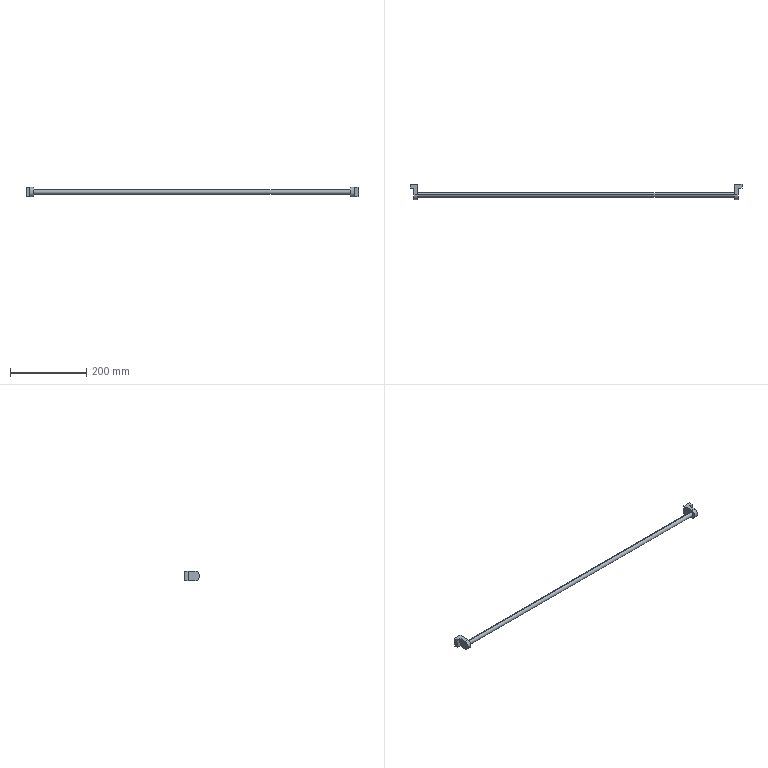Component | SolidWorks | D014-1 | 2 solids | 22 faces | box 869 x 40 x 25 mm | volume 117416 mm3 | plane 16 | cylinder 6 | commonest cylinder face diameters 12 x4 25 x2
build123d program:
from build123d import *

# Parameters (mm, degrees)
SKETCH1_W           = 40
SKETCH1_H           = 25
BOSS_EXTRUDE1_DEPTH = 10
FILLET1_RADIUS      = 12.5
FILLET1_LENGTH      = 10
SKETCH2_R           = 6
CUT_EXTRUDE1_DEPTH  = 2
SKETCH3_R           = 6
BOSS_EXTRUDE2_DEPTH = 831
BOSS_EXTRUDE3_START = 10
BOSS_EXTRUDE3_DEPTH = 10
SKETCH5_W           = 25
SKETCH5_H           = 10
BOSS_EXTRUDE4_DEPTH = 10
SKETCH6_W           = 25
SKETCH6_H           = 10
BOSS_EXTRUDE5_DEPTH = 10


with BuildPart() as part:
    # Sketch1 → Boss-Extrude1 (new body)
    with BuildSketch(Plane(origin=(0, 0, 0), x_dir=(1, 0, 0), z_dir=(0, 1, 0))):
        with Locations((20, 12.5)):
            Rectangle(SKETCH1_W, SKETCH1_H)
    extrude(amount=BOSS_EXTRUDE1_DEPTH)

    # Fillet1: full round fillet: the end face becomes a half cylinder, R = half its width
    fillet1_face = Plane((40, 5, -12.5), x_dir=(0, 1, 0), z_dir=(1, 0, 0))  # on the end face: x along it, z out of the body
    fillet1_slab = fillet1_face.offset(-FILLET1_RADIUS / 2) * Box(FILLET1_LENGTH, 2 * FILLET1_RADIUS, FILLET1_RADIUS, mode=Mode.PRIVATE)  # the body's end, R deep
    fillet1_round = Plane((27.5, 5, -12.5), x_dir=(1, 0, 0), z_dir=(0, 1, 0)) * Cylinder(FILLET1_RADIUS, FILLET1_LENGTH, mode=Mode.PRIVATE)  # its axis R under the face
    add(fillet1_slab - fillet1_round, mode=Mode.SUBTRACT)

    # Sketch2 → Cut-Extrude1 (cut)
    with BuildSketch(Plane(origin=(0, 10, 0), x_dir=(1, 0, 0), z_dir=(0, 1, 0))):
        with Locations(Location((27.5, 12.5, 0), (0, 0, 270))):
            Circle(SKETCH2_R)
    extrude(amount=-CUT_EXTRUDE1_DEPTH, mode=Mode.SUBTRACT)

    # Sketch6 → Boss-Extrude5 (add)
    with BuildSketch(Plane.ZY):
        with Locations((-12.5, -5)):
            Rectangle(SKETCH6_W, SKETCH6_H)
    extrude(amount=-BOSS_EXTRUDE5_DEPTH)


with BuildPart() as body_2:
    # Sketch3 → Boss-Extrude2 (new body)
    with BuildSketch(Plane(origin=(0, 8, 0), x_dir=(1, 0, 0), z_dir=(0, 1, 0))):
        with Locations(Location((27.5, 12.5, 0), (0, 0, 270))):
            Circle(SKETCH3_R)
    extrude(amount=BOSS_EXTRUDE2_DEPTH)

    # Sketch4 → Boss-Extrude3 (add)
    with BuildSketch(Plane(origin=(0, 839, 0), x_dir=(1, 0, 0), z_dir=(0, 1, 0)).offset(BOSS_EXTRUDE3_START)):
        with BuildLine():
            Line((0, 0), (27.5, 0))
            ThreePointArc((27.5, 0), (40, 12.5), (27.5, 25))
            Line((27.5, 25), (0, 25))
            Line((0, 25), (0, 0))
        make_face()
    extrude(amount=-BOSS_EXTRUDE3_DEPTH)

    # Sketch5 → Boss-Extrude4 (add)
    with BuildSketch(Plane.ZY):
        with Locations((-12.5, 854)):
            Rectangle(SKETCH5_W, SKETCH5_H)
    extrude(amount=-BOSS_EXTRUDE4_DEPTH)


solid = Compound([part.part, body_2.part])

# Placed as in the assembly
solid = solid.moved(Location((859, -60, -101.268), (180, 0, 90)))
STEP:
#1=COLOUR_RGB('',0.7922,0.8196,0.9333);
#2=FILL_AREA_STYLE_COLOUR('',#1);
#3=FILL_AREA_STYLE('',(#2));
#4=SURFACE_STYLE_FILL_AREA(#3);
#5=SURFACE_SIDE_STYLE('',(#4));
#6=SURFACE_STYLE_USAGE(.BOTH.,#5);
#7=PRESENTATION_STYLE_ASSIGNMENT((#6));
#8=CARTESIAN_POINT('',(33.504,-3.445,-3.259));
#9=VERTEX_POINT('',#8);
#10=CARTESIAN_POINT('',(33.504,-3.445,-3.731));
#11=VERTEX_POINT('',#10);
#12=CARTESIAN_POINT('',(33.504,-3.445,-3.495));
#13=DIRECTION('',(-1.,0.,0.));
#14=DIRECTION('',(0.,0.,-1.));
#15=AXIS2_PLACEMENT_3D('',#12,#13,#14);
#16=CIRCLE('',#15,0.2362);
#17=EDGE_CURVE('',#9,#11,#16,.T.);
#18=ORIENTED_EDGE('',*,*,#17,.F.);
#19=CARTESIAN_POINT('',(33.425,-3.445,-3.259));
#20=VERTEX_POINT('',#19);
#21=CARTESIAN_POINT('',(33.504,-3.445,-3.259));
#22=DIRECTION('',(-1.,0.,0.));
#23=VECTOR('',#22,39.37);
#24=LINE('',#21,#23);
#25=EDGE_CURVE('',#9,#20,#24,.T.);
#26=ORIENTED_EDGE('',*,*,#25,.T.);
#27=CARTESIAN_POINT('',(33.425,-3.445,-3.731));
#28=VERTEX_POINT('',#27);
#29=CARTESIAN_POINT('',(33.425,-3.445,-3.495));
#30=DIRECTION('',(-1.,0.,0.));
#31=DIRECTION('',(0.,0.,-1.));
#32=AXIS2_PLACEMENT_3D('',#29,#30,#31);
#33=CIRCLE('',#32,0.2362);
#34=EDGE_CURVE('',#20,#28,#33,.T.);
#35=ORIENTED_EDGE('',*,*,#34,.T.);
#36=CARTESIAN_POINT('',(33.504,-3.445,-3.731));
#37=DIRECTION('',(-1.,0.,0.));
#38=VECTOR('',#37,39.37);
#39=LINE('',#36,#38);
#40=EDGE_CURVE('',#11,#28,#39,.T.);
#41=ORIENTED_EDGE('',*,*,#40,.F.);
#42=EDGE_LOOP('',(#18,#26,#35,#41));
#43=FACE_OUTER_BOUND('',#42,.T.);
#44=CARTESIAN_POINT('',(33.504,-3.445,-3.495));
#45=DIRECTION('',(-1.,0.,0.));
#46=DIRECTION('',(0.,0.,-1.));
#47=AXIS2_PLACEMENT_3D('',#44,#45,#46);
#48=CYLINDRICAL_SURFACE('',#47,0.2362);
#49=ADVANCED_FACE('',(#43),#48,.F.);
#50=CARTESIAN_POINT('',(33.819,-2.756,-3.987));
#51=VERTEX_POINT('',#50);
#52=CARTESIAN_POINT('',(33.819,-3.445,-3.987));
#53=VERTEX_POINT('',#52);
#54=CARTESIAN_POINT('',(33.819,-2.362,-3.987));
#55=DIRECTION('',(-0.,-1.,-0.));
#56=VECTOR('',#55,39.37);
#57=LINE('',#54,#56);
#58=EDGE_CURVE('',#51,#53,#57,.T.);
#59=ORIENTED_EDGE('',*,*,#58,.F.);
#60=CARTESIAN_POINT('',(33.819,-2.756,-3.003));
#61=VERTEX_POINT('',#60);
#62=CARTESIAN_POINT('',(33.819,-2.756,-3.003));
#63=DIRECTION('',(0.,-0.,1.));
#64=VECTOR('',#63,39.37);
#65=LINE('',#62,#64);
#66=EDGE_CURVE('',#51,#61,#65,.T.);
#67=ORIENTED_EDGE('',*,*,#66,.T.);
#68=CARTESIAN_POINT('',(33.819,-3.445,-3.003));
#69=VERTEX_POINT('',#68);
#70=CARTESIAN_POINT('',(33.819,-2.362,-3.003));
#71=DIRECTION('',(0.,1.,0.));
#72=VECTOR('',#71,39.37);
#73=LINE('',#70,#72);
#74=EDGE_CURVE('',#69,#61,#73,.T.);
#75=ORIENTED_EDGE('',*,*,#74,.F.);
#76=CARTESIAN_POINT('',(33.819,-3.445,-3.495));
#77=DIRECTION('',(1.,-0.,-0.));
#78=DIRECTION('',(0.,-0.,1.));
#79=AXIS2_PLACEMENT_3D('',#76,#77,#78);
#80=CIRCLE('',#79,0.4921);
#81=EDGE_CURVE('',#69,#53,#80,.T.);
#82=ORIENTED_EDGE('',*,*,#81,.T.);
#83=EDGE_LOOP('',(#59,#67,#75,#82));
#84=FACE_OUTER_BOUND('',#83,.T.);
#85=CARTESIAN_POINT('',(33.819,-2.362,-3.987));
#86=DIRECTION('',(1.,-0.,-0.));
#87=DIRECTION('',(0.,-0.,1.));
#88=AXIS2_PLACEMENT_3D('',#85,#86,#87);
#89=PLANE('',#88);
#90=ADVANCED_FACE('',(#84),#89,.T.);
#91=CARTESIAN_POINT('',(33.425,-3.445,-3.987));
#92=VERTEX_POINT('',#91);
#93=CARTESIAN_POINT('',(33.425,-3.445,-3.987));
#94=DIRECTION('',(-1.,0.,0.));
#95=VECTOR('',#94,39.37);
#96=LINE('',#93,#95);
#97=EDGE_CURVE('',#53,#92,#96,.T.);
#98=ORIENTED_EDGE('',*,*,#97,.F.);
#99=ORIENTED_EDGE('',*,*,#81,.F.);
#100=CARTESIAN_POINT('',(33.425,-3.445,-3.003));
#101=VERTEX_POINT('',#100);
#102=CARTESIAN_POINT('',(33.425,-3.445,-3.003));
#103=DIRECTION('',(1.,-0.,-0.));
#104=VECTOR('',#103,39.37);
#105=LINE('',#102,#104);
#106=EDGE_CURVE('',#101,#69,#105,.T.);
#107=ORIENTED_EDGE('',*,*,#106,.F.);
#108=CARTESIAN_POINT('',(33.425,-3.445,-3.495));
#109=DIRECTION('',(-1.,0.,0.));
#110=DIRECTION('',(0.,-0.,1.));
#111=AXIS2_PLACEMENT_3D('',#108,#109,#110);
#112=CIRCLE('',#111,0.4921);
#113=EDGE_CURVE('',#92,#101,#112,.T.);
#114=ORIENTED_EDGE('',*,*,#113,.F.);
#115=EDGE_LOOP('',(#98,#99,#107,#114));
#116=FACE_OUTER_BOUND('',#115,.T.);
#117=CARTESIAN_POINT('',(33.819,-3.445,-3.495));
#118=DIRECTION('',(1.,-0.,-0.));
#119=DIRECTION('',(0.,-0.,1.));
#120=AXIS2_PLACEMENT_3D('',#117,#118,#119);
#121=CYLINDRICAL_SURFACE('',#120,0.4921);
#122=ADVANCED_FACE('',(#116),#121,.T.);
#123=CARTESIAN_POINT('',(33.425,-2.362,-3.003));
#124=VERTEX_POINT('',#123);
#125=CARTESIAN_POINT('',(34.213,-2.362,-3.003));
#126=VERTEX_POINT('',#125);
#127=CARTESIAN_POINT('',(33.425,-2.362,-3.003));
#128=DIRECTION('',(1.,-0.,-0.));
#129=VECTOR('',#128,39.37);
#130=LINE('',#127,#129);
#131=EDGE_CURVE('',#124,#126,#130,.T.);
#132=ORIENTED_EDGE('',*,*,#131,.T.);
#133=CARTESIAN_POINT('',(34.213,-2.362,-3.987));
#134=VERTEX_POINT('',#133);
#135=CARTESIAN_POINT('',(34.213,-2.362,-3.003));
#136=DIRECTION('',(-0.,0.,-1.));
#137=VECTOR('',#136,39.37);
#138=LINE('',#135,#137);
#139=EDGE_CURVE('',#126,#134,#138,.T.);
#140=ORIENTED_EDGE('',*,*,#139,.T.);
#141=CARTESIAN_POINT('',(33.425,-2.362,-3.987));
#142=VERTEX_POINT('',#141);
#143=CARTESIAN_POINT('',(33.425,-2.362,-3.987));
#144=DIRECTION('',(1.,-0.,-0.));
#145=VECTOR('',#144,39.37);
#146=LINE('',#143,#145);
#147=EDGE_CURVE('',#142,#134,#146,.T.);
#148=ORIENTED_EDGE('',*,*,#147,.F.);
#149=CARTESIAN_POINT('',(33.425,-2.362,-3.987));
#150=DIRECTION('',(-0.,0.,-1.));
#151=VECTOR('',#150,39.37);
#152=LINE('',#149,#151);
#153=EDGE_CURVE('',#124,#142,#152,.T.);
#154=ORIENTED_EDGE('',*,*,#153,.F.);
#155=EDGE_LOOP('',(#132,#140,#148,#154));
#156=FACE_OUTER_BOUND('',#155,.T.);
#157=CARTESIAN_POINT('',(33.425,-2.362,-3.987));
#158=DIRECTION('',(-0.,-1.,-0.));
#159=DIRECTION('',(0.,-0.,1.));
#160=AXIS2_PLACEMENT_3D('',#157,#158,#159);
#161=PLANE('',#160);
#162=ADVANCED_FACE('',(#156),#161,.F.);
#163=ORIENTED_EDGE('',*,*,#147,.T.);
#164=CARTESIAN_POINT('',(34.213,-2.756,-3.987));
#165=VERTEX_POINT('',#164);
#166=CARTESIAN_POINT('',(34.213,-2.756,-3.987));
#167=DIRECTION('',(0.,1.,0.));
#168=VECTOR('',#167,39.37);
#169=LINE('',#166,#168);
#170=EDGE_CURVE('',#165,#134,#169,.T.);
#171=ORIENTED_EDGE('',*,*,#170,.F.);
#172=CARTESIAN_POINT('',(33.819,-2.756,-3.987));
#173=DIRECTION('',(-1.,0.,0.));
#174=VECTOR('',#173,39.37);
#175=LINE('',#172,#174);
#176=EDGE_CURVE('',#165,#51,#175,.T.);
#177=ORIENTED_EDGE('',*,*,#176,.T.);
#178=ORIENTED_EDGE('',*,*,#58,.T.);
#179=ORIENTED_EDGE('',*,*,#97,.T.);
#180=CARTESIAN_POINT('',(33.425,-2.362,-3.987));
#181=DIRECTION('',(-0.,-1.,-0.));
#182=VECTOR('',#181,39.37);
#183=LINE('',#180,#182);
#184=EDGE_CURVE('',#142,#92,#183,.T.);
#185=ORIENTED_EDGE('',*,*,#184,.F.);
#186=EDGE_LOOP('',(#163,#171,#177,#178,#179,#185));
#187=FACE_OUTER_BOUND('',#186,.T.);
#188=CARTESIAN_POINT('',(33.425,-2.362,-3.987));
#189=DIRECTION('',(0.,-0.,1.));
#190=DIRECTION('',(0.,1.,0.));
#191=AXIS2_PLACEMENT_3D('',#188,#189,#190);
#192=PLANE('',#191);
#193=ADVANCED_FACE('',(#187),#192,.F.);
#194=CARTESIAN_POINT('',(33.425,-2.362,-3.003));
#195=DIRECTION('',(0.,1.,0.));
#196=VECTOR('',#195,39.37);
#197=LINE('',#194,#196);
#198=EDGE_CURVE('',#101,#124,#197,.T.);
#199=ORIENTED_EDGE('',*,*,#198,.F.);
#200=ORIENTED_EDGE('',*,*,#106,.T.);
#201=ORIENTED_EDGE('',*,*,#74,.T.);
#202=CARTESIAN_POINT('',(34.213,-2.756,-3.003));
#203=VERTEX_POINT('',#202);
#204=CARTESIAN_POINT('',(33.819,-2.756,-3.003));
#205=DIRECTION('',(1.,-0.,-0.));
#206=VECTOR('',#205,39.37);
#207=LINE('',#204,#206);
#208=EDGE_CURVE('',#61,#203,#207,.T.);
#209=ORIENTED_EDGE('',*,*,#208,.T.);
#210=CARTESIAN_POINT('',(34.213,-2.756,-3.003));
#211=DIRECTION('',(0.,1.,0.));
#212=VECTOR('',#211,39.37);
#213=LINE('',#210,#212);
#214=EDGE_CURVE('',#203,#126,#213,.T.);
#215=ORIENTED_EDGE('',*,*,#214,.T.);
#216=ORIENTED_EDGE('',*,*,#131,.F.);
#217=EDGE_LOOP('',(#199,#200,#201,#209,#215,#216));
#218=FACE_OUTER_BOUND('',#217,.T.);
#219=CARTESIAN_POINT('',(33.425,-2.362,-3.003));
#220=DIRECTION('',(-0.,0.,-1.));
#221=DIRECTION('',(-0.,-1.,-0.));
#222=AXIS2_PLACEMENT_3D('',#219,#220,#221);
#223=PLANE('',#222);
#224=ADVANCED_FACE('',(#218),#223,.F.);
#225=CARTESIAN_POINT('',(33.425,-3.445,-3.495));
#226=DIRECTION('',(-1.,0.,0.));
#227=DIRECTION('',(0.,0.,-1.));
#228=AXIS2_PLACEMENT_3D('',#225,#226,#227);
#229=CIRCLE('',#228,0.2362);
#230=EDGE_CURVE('',#28,#20,#229,.T.);
#231=ORIENTED_EDGE('',*,*,#230,.F.);
#232=ORIENTED_EDGE('',*,*,#34,.F.);
#233=EDGE_LOOP('',(#231,#232));
#234=FACE_BOUND('',#233,.T.);
#235=ORIENTED_EDGE('',*,*,#184,.T.);
#236=ORIENTED_EDGE('',*,*,#113,.T.);
#237=ORIENTED_EDGE('',*,*,#198,.T.);
#238=ORIENTED_EDGE('',*,*,#153,.T.);
#239=EDGE_LOOP('',(#235,#236,#237,#238));
#240=FACE_OUTER_BOUND('',#239,.T.);
#241=CARTESIAN_POINT('',(33.425,-2.362,-3.987));
#242=DIRECTION('',(1.,-0.,-0.));
#243=DIRECTION('',(0.,-0.,1.));
#244=AXIS2_PLACEMENT_3D('',#241,#242,#243);
#245=PLANE('',#244);
#246=ADVANCED_FACE('',(#234,#240),#245,.F.);
#247=ORIENTED_EDGE('',*,*,#25,.F.);
#248=CARTESIAN_POINT('',(33.504,-3.445,-3.495));
#249=DIRECTION('',(-1.,0.,0.));
#250=DIRECTION('',(0.,0.,-1.));
#251=AXIS2_PLACEMENT_3D('',#248,#249,#250);
#252=CIRCLE('',#251,0.2362);
#253=EDGE_CURVE('',#11,#9,#252,.T.);
#254=ORIENTED_EDGE('',*,*,#253,.F.);
#255=ORIENTED_EDGE('',*,*,#40,.T.);
#256=ORIENTED_EDGE('',*,*,#230,.T.);
#257=EDGE_LOOP('',(#247,#254,#255,#256));
#258=FACE_OUTER_BOUND('',#257,.T.);
#259=CARTESIAN_POINT('',(33.504,-3.445,-3.495));
#260=DIRECTION('',(-1.,0.,0.));
#261=DIRECTION('',(0.,0.,-1.));
#262=AXIS2_PLACEMENT_3D('',#259,#260,#261);
#263=CYLINDRICAL_SURFACE('',#262,0.2362);
#264=ADVANCED_FACE('',(#258),#263,.F.);
#265=ORIENTED_EDGE('',*,*,#253,.T.);
#266=ORIENTED_EDGE('',*,*,#17,.T.);
#267=EDGE_LOOP('',(#265,#266));
#268=FACE_OUTER_BOUND('',#267,.T.);
#269=CARTESIAN_POINT('',(33.504,-3.445,-3.495));
#270=DIRECTION('',(-1.,0.,0.));
#271=DIRECTION('',(-0.,0.,-1.));
#272=AXIS2_PLACEMENT_3D('',#269,#270,#271);
#273=PLANE('',#272);
#274=ADVANCED_FACE('',(#268),#273,.T.);
#275=ORIENTED_EDGE('',*,*,#139,.F.);
#276=ORIENTED_EDGE('',*,*,#214,.F.);
#277=CARTESIAN_POINT('',(34.213,-2.756,-3.003));
#278=DIRECTION('',(-0.,0.,-1.));
#279=VECTOR('',#278,39.37);
#280=LINE('',#277,#279);
#281=EDGE_CURVE('',#203,#165,#280,.T.);
#282=ORIENTED_EDGE('',*,*,#281,.T.);
#283=ORIENTED_EDGE('',*,*,#170,.T.);
#284=EDGE_LOOP('',(#275,#276,#282,#283));
#285=FACE_OUTER_BOUND('',#284,.T.);
#286=CARTESIAN_POINT('',(34.213,-2.756,-3.003));
#287=DIRECTION('',(1.,-0.,-0.));
#288=DIRECTION('',(0.,-0.,1.));
#289=AXIS2_PLACEMENT_3D('',#286,#287,#288);
#290=PLANE('',#289);
#291=ADVANCED_FACE('',(#285),#290,.T.);
#292=ORIENTED_EDGE('',*,*,#208,.F.);
#293=ORIENTED_EDGE('',*,*,#66,.F.);
#294=ORIENTED_EDGE('',*,*,#176,.F.);
#295=ORIENTED_EDGE('',*,*,#281,.F.);
#296=EDGE_LOOP('',(#292,#293,#294,#295));
#297=FACE_OUTER_BOUND('',#296,.T.);
#298=CARTESIAN_POINT('',(33.819,-2.756,-3.987));
#299=DIRECTION('',(0.,1.,0.));
#300=DIRECTION('',(-0.,0.,-1.));
#301=AXIS2_PLACEMENT_3D('',#298,#299,#300);
#302=PLANE('',#301);
#303=ADVANCED_FACE('',(#297),#302,.F.);
#304=CLOSED_SHELL('',(#49,#90,#122,#162,#193,#224,#246,#264,#274,#291,#303));
#305=MANIFOLD_SOLID_BREP('',#304);
#306=STYLED_ITEM('',(#7),#305);
#307=(LENGTH_UNIT()NAMED_UNIT(*)SI_UNIT($,.METRE.));
#308=LENGTH_MEASURE_WITH_UNIT(LENGTH_MEASURE(0.0254),#307);
#309=DIMENSIONAL_EXPONENTS(1.,0.,0.,0.,0.,0.,0.);
#310=(CONVERSION_BASED_UNIT('',#308)LENGTH_UNIT()NAMED_UNIT(#309));
#311=UNCERTAINTY_MEASURE_WITH_UNIT(LENGTH_MEASURE(0.00001),#310,'','');
#312=(NAMED_UNIT(*)PLANE_ANGLE_UNIT()SI_UNIT($,.RADIAN.));
#313=(NAMED_UNIT(*)SI_UNIT($,.STERADIAN.)SOLID_ANGLE_UNIT());
#314=(GEOMETRIC_REPRESENTATION_CONTEXT(3)GLOBAL_UNCERTAINTY_ASSIGNED_CONTEXT((#311))GLOBAL_UNIT_ASSIGNED_CONTEXT((#310,#312,#313))REPRESENTATION_CONTEXT('',''));
#315=MECHANICAL_DESIGN_GEOMETRIC_PRESENTATION_REPRESENTATION('',(#306),#314);
#316=COLOUR_RGB('',0.7922,0.8196,0.9333);
#317=FILL_AREA_STYLE_COLOUR('',#316);
#318=FILL_AREA_STYLE('',(#317));
#319=SURFACE_STYLE_FILL_AREA(#318);
#320=SURFACE_SIDE_STYLE('',(#319));
#321=SURFACE_STYLE_USAGE(.BOTH.,#320);
#322=PRESENTATION_STYLE_ASSIGNMENT((#321));
#323=CARTESIAN_POINT('',(0.7874,-3.445,-3.731));
#324=VERTEX_POINT('',#323);
#325=CARTESIAN_POINT('',(0.7874,-3.445,-3.259));
#326=VERTEX_POINT('',#325);
#327=CARTESIAN_POINT('',(0.7874,-3.445,-3.495));
#328=DIRECTION('',(-1.,0.,0.));
#329=DIRECTION('',(0.,0.,-1.));
#330=AXIS2_PLACEMENT_3D('',#327,#328,#329);
#331=CIRCLE('',#330,0.2362);
#332=EDGE_CURVE('',#324,#326,#331,.T.);
#333=ORIENTED_EDGE('',*,*,#332,.F.);
#334=CARTESIAN_POINT('',(33.504,-3.445,-3.731));
#335=VERTEX_POINT('',#334);
#336=CARTESIAN_POINT('',(0.7874,-3.445,-3.731));
#337=DIRECTION('',(1.,-0.,-0.));
#338=VECTOR('',#337,39.37);
#339=LINE('',#336,#338);
#340=EDGE_CURVE('',#324,#335,#339,.T.);
#341=ORIENTED_EDGE('',*,*,#340,.T.);
#342=CARTESIAN_POINT('',(33.504,-3.445,-3.259));
#343=VERTEX_POINT('',#342);
#344=CARTESIAN_POINT('',(33.504,-3.445,-3.495));
#345=DIRECTION('',(-1.,0.,0.));
#346=DIRECTION('',(0.,0.,-1.));
#347=AXIS2_PLACEMENT_3D('',#344,#345,#346);
#348=CIRCLE('',#347,0.2362);
#349=EDGE_CURVE('',#335,#343,#348,.T.);
#350=ORIENTED_EDGE('',*,*,#349,.T.);
#351=CARTESIAN_POINT('',(0.7874,-3.445,-3.259));
#352=DIRECTION('',(1.,-0.,-0.));
#353=VECTOR('',#352,39.37);
#354=LINE('',#351,#353);
#355=EDGE_CURVE('',#326,#343,#354,.T.);
#356=ORIENTED_EDGE('',*,*,#355,.F.);
#357=EDGE_LOOP('',(#333,#341,#350,#356));
#358=FACE_OUTER_BOUND('',#357,.T.);
#359=CARTESIAN_POINT('',(0.7874,-3.445,-3.495));
#360=DIRECTION('',(1.,-0.,-0.));
#361=DIRECTION('',(0.,-0.,1.));
#362=AXIS2_PLACEMENT_3D('',#359,#360,#361);
#363=CYLINDRICAL_SURFACE('',#362,0.2362);
#364=ADVANCED_FACE('',(#358),#363,.T.);
#365=CARTESIAN_POINT('',(0.3937,-3.445,-3.003));
#366=VERTEX_POINT('',#365);
#367=CARTESIAN_POINT('',(0.3937,-2.756,-3.003));
#368=VERTEX_POINT('',#367);
#369=CARTESIAN_POINT('',(0.3937,-3.445,-3.003));
#370=DIRECTION('',(0.,1.,0.));
#371=VECTOR('',#370,39.37);
#372=LINE('',#369,#371);
#373=EDGE_CURVE('',#366,#368,#372,.T.);
#374=ORIENTED_EDGE('',*,*,#373,.T.);
#375=CARTESIAN_POINT('',(0.3937,-2.756,-3.987));
#376=VERTEX_POINT('',#375);
#377=CARTESIAN_POINT('',(0.3937,-2.756,-3.003));
#378=DIRECTION('',(-0.,0.,-1.));
#379=VECTOR('',#378,39.37);
#380=LINE('',#377,#379);
#381=EDGE_CURVE('',#368,#376,#380,.T.);
#382=ORIENTED_EDGE('',*,*,#381,.T.);
#383=CARTESIAN_POINT('',(0.3937,-3.445,-3.987));
#384=VERTEX_POINT('',#383);
#385=CARTESIAN_POINT('',(0.3937,-2.362,-3.987));
#386=DIRECTION('',(-0.,-1.,-0.));
#387=VECTOR('',#386,39.37);
#388=LINE('',#385,#387);
#389=EDGE_CURVE('',#376,#384,#388,.T.);
#390=ORIENTED_EDGE('',*,*,#389,.T.);
#391=CARTESIAN_POINT('',(0.3937,-3.445,-3.495));
#392=DIRECTION('',(-1.,0.,0.));
#393=DIRECTION('',(0.,0.,-1.));
#394=AXIS2_PLACEMENT_3D('',#391,#392,#393);
#395=CIRCLE('',#394,0.4921);
#396=EDGE_CURVE('',#384,#366,#395,.T.);
#397=ORIENTED_EDGE('',*,*,#396,.T.);
#398=EDGE_LOOP('',(#374,#382,#390,#397));
#399=FACE_OUTER_BOUND('',#398,.T.);
#400=CARTESIAN_POINT('',(0.3937,-3.445,-3.495));
#401=DIRECTION('',(-1.,0.,0.));
#402=DIRECTION('',(-0.,0.,-1.));
#403=AXIS2_PLACEMENT_3D('',#400,#401,#402);
#404=PLANE('',#403);
#405=ADVANCED_FACE('',(#399),#404,.T.);
#406=ORIENTED_EDGE('',*,*,#340,.F.);
#407=CARTESIAN_POINT('',(0.7874,-3.445,-3.495));
#408=DIRECTION('',(-1.,0.,0.));
#409=DIRECTION('',(0.,0.,-1.));
#410=AXIS2_PLACEMENT_3D('',#407,#408,#409);
#411=CIRCLE('',#410,0.2362);
#412=EDGE_CURVE('',#326,#324,#411,.T.);
#413=ORIENTED_EDGE('',*,*,#412,.F.);
#414=ORIENTED_EDGE('',*,*,#355,.T.);
#415=CARTESIAN_POINT('',(33.504,-3.445,-3.495));
#416=DIRECTION('',(-1.,0.,0.));
#417=DIRECTION('',(0.,0.,-1.));
#418=AXIS2_PLACEMENT_3D('',#415,#416,#417);
#419=CIRCLE('',#418,0.2362);
#420=EDGE_CURVE('',#343,#335,#419,.T.);
#421=ORIENTED_EDGE('',*,*,#420,.T.);
#422=EDGE_LOOP('',(#406,#413,#414,#421));
#423=FACE_OUTER_BOUND('',#422,.T.);
#424=CARTESIAN_POINT('',(0.7874,-3.445,-3.495));
#425=DIRECTION('',(1.,-0.,-0.));
#426=DIRECTION('',(0.,-0.,1.));
#427=AXIS2_PLACEMENT_3D('',#424,#425,#426);
#428=CYLINDRICAL_SURFACE('',#427,0.2362);
#429=ADVANCED_FACE('',(#423),#428,.T.);
#430=ORIENTED_EDGE('',*,*,#420,.F.);
#431=ORIENTED_EDGE('',*,*,#349,.F.);
#432=EDGE_LOOP('',(#430,#431));
#433=FACE_OUTER_BOUND('',#432,.T.);
#434=CARTESIAN_POINT('',(33.504,-3.445,-3.495));
#435=DIRECTION('',(-1.,0.,0.));
#436=DIRECTION('',(-0.,0.,-1.));
#437=AXIS2_PLACEMENT_3D('',#434,#435,#436);
#438=PLANE('',#437);
#439=ADVANCED_FACE('',(#433),#438,.F.);
#440=CARTESIAN_POINT('',(0.7874,-2.362,-3.003));
#441=VERTEX_POINT('',#440);
#442=CARTESIAN_POINT('',(0.7874,-2.362,-3.987));
#443=VERTEX_POINT('',#442);
#444=CARTESIAN_POINT('',(0.7874,-2.362,-3.003));
#445=DIRECTION('',(-0.,0.,-1.));
#446=VECTOR('',#445,39.37);
#447=LINE('',#444,#446);
#448=EDGE_CURVE('',#441,#443,#447,.T.);
#449=ORIENTED_EDGE('',*,*,#448,.T.);
#450=CARTESIAN_POINT('',(-0.,-2.362,-3.987));
#451=VERTEX_POINT('',#450);
#452=CARTESIAN_POINT('',(0.3937,-2.362,-3.987));
#453=DIRECTION('',(1.,-0.,-0.));
#454=VECTOR('',#453,39.37);
#455=LINE('',#452,#454);
#456=EDGE_CURVE('',#451,#443,#455,.T.);
#457=ORIENTED_EDGE('',*,*,#456,.F.);
#458=CARTESIAN_POINT('',(-0.,-2.362,-3.003));
#459=VERTEX_POINT('',#458);
#460=CARTESIAN_POINT('',(-0.,-2.362,-3.003));
#461=DIRECTION('',(0.,-0.,1.));
#462=VECTOR('',#461,39.37);
#463=LINE('',#460,#462);
#464=EDGE_CURVE('',#451,#459,#463,.T.);
#465=ORIENTED_EDGE('',*,*,#464,.T.);
#466=CARTESIAN_POINT('',(0.3937,-2.362,-3.003));
#467=DIRECTION('',(1.,-0.,-0.));
#468=VECTOR('',#467,39.37);
#469=LINE('',#466,#468);
#470=EDGE_CURVE('',#459,#441,#469,.T.);
#471=ORIENTED_EDGE('',*,*,#470,.T.);
#472=EDGE_LOOP('',(#449,#457,#465,#471));
#473=FACE_OUTER_BOUND('',#472,.T.);
#474=CARTESIAN_POINT('',(0.3937,-2.362,-3.003));
#475=DIRECTION('',(-0.,-1.,-0.));
#476=DIRECTION('',(0.,-0.,1.));
#477=AXIS2_PLACEMENT_3D('',#474,#475,#476);
#478=PLANE('',#477);
#479=ADVANCED_FACE('',(#473),#478,.F.);
#480=CARTESIAN_POINT('',(0.7874,-3.445,-3.987));
#481=VERTEX_POINT('',#480);
#482=CARTESIAN_POINT('',(0.7874,-2.362,-3.987));
#483=DIRECTION('',(-0.,-1.,-0.));
#484=VECTOR('',#483,39.37);
#485=LINE('',#482,#484);
#486=EDGE_CURVE('',#443,#481,#485,.T.);
#487=ORIENTED_EDGE('',*,*,#486,.T.);
#488=CARTESIAN_POINT('',(0.3937,-3.445,-3.987));
#489=DIRECTION('',(1.,-0.,-0.));
#490=VECTOR('',#489,39.37);
#491=LINE('',#488,#490);
#492=EDGE_CURVE('',#384,#481,#491,.T.);
#493=ORIENTED_EDGE('',*,*,#492,.F.);
#494=ORIENTED_EDGE('',*,*,#389,.F.);
#495=CARTESIAN_POINT('',(-0.,-2.756,-3.987));
#496=VERTEX_POINT('',#495);
#497=CARTESIAN_POINT('',(0.3937,-2.756,-3.987));
#498=DIRECTION('',(-1.,0.,0.));
#499=VECTOR('',#498,39.37);
#500=LINE('',#497,#499);
#501=EDGE_CURVE('',#376,#496,#500,.T.);
#502=ORIENTED_EDGE('',*,*,#501,.T.);
#503=CARTESIAN_POINT('',(-0.,-2.756,-3.987));
#504=DIRECTION('',(0.,1.,0.));
#505=VECTOR('',#504,39.37);
#506=LINE('',#503,#505);
#507=EDGE_CURVE('',#496,#451,#506,.T.);
#508=ORIENTED_EDGE('',*,*,#507,.T.);
#509=ORIENTED_EDGE('',*,*,#456,.T.);
#510=EDGE_LOOP('',(#487,#493,#494,#502,#508,#509));
#511=FACE_OUTER_BOUND('',#510,.T.);
#512=CARTESIAN_POINT('',(0.3937,-2.362,-3.987));
#513=DIRECTION('',(0.,-0.,1.));
#514=DIRECTION('',(0.,1.,0.));
#515=AXIS2_PLACEMENT_3D('',#512,#513,#514);
#516=PLANE('',#515);
#517=ADVANCED_FACE('',(#511),#516,.F.);
#518=CARTESIAN_POINT('',(0.7874,-3.445,-3.003));
#519=VERTEX_POINT('',#518);
#520=CARTESIAN_POINT('',(0.7874,-3.445,-3.495));
#521=DIRECTION('',(-1.,0.,0.));
#522=DIRECTION('',(0.,0.,-1.));
#523=AXIS2_PLACEMENT_3D('',#520,#521,#522);
#524=CIRCLE('',#523,0.4921);
#525=EDGE_CURVE('',#481,#519,#524,.T.);
#526=ORIENTED_EDGE('',*,*,#525,.T.);
#527=CARTESIAN_POINT('',(0.3937,-3.445,-3.003));
#528=DIRECTION('',(1.,-0.,-0.));
#529=VECTOR('',#528,39.37);
#530=LINE('',#527,#529);
#531=EDGE_CURVE('',#366,#519,#530,.T.);
#532=ORIENTED_EDGE('',*,*,#531,.F.);
#533=ORIENTED_EDGE('',*,*,#396,.F.);
#534=ORIENTED_EDGE('',*,*,#492,.T.);
#535=EDGE_LOOP('',(#526,#532,#533,#534));
#536=FACE_OUTER_BOUND('',#535,.T.);
#537=CARTESIAN_POINT('',(0.3937,-3.445,-3.495));
#538=DIRECTION('',(1.,-0.,-0.));
#539=DIRECTION('',(0.,-0.,1.));
#540=AXIS2_PLACEMENT_3D('',#537,#538,#539);
#541=CYLINDRICAL_SURFACE('',#540,0.4921);
#542=ADVANCED_FACE('',(#536),#541,.T.);
#543=CARTESIAN_POINT('',(0.7874,-3.445,-3.003));
#544=DIRECTION('',(0.,1.,0.));
#545=VECTOR('',#544,39.37);
#546=LINE('',#543,#545);
#547=EDGE_CURVE('',#519,#441,#546,.T.);
#548=ORIENTED_EDGE('',*,*,#547,.T.);
#549=ORIENTED_EDGE('',*,*,#470,.F.);
#550=CARTESIAN_POINT('',(-0.,-2.756,-3.003));
#551=VERTEX_POINT('',#550);
#552=CARTESIAN_POINT('',(-0.,-2.756,-3.003));
#553=DIRECTION('',(0.,1.,0.));
#554=VECTOR('',#553,39.37);
#555=LINE('',#552,#554);
#556=EDGE_CURVE('',#551,#459,#555,.T.);
#557=ORIENTED_EDGE('',*,*,#556,.F.);
#558=CARTESIAN_POINT('',(0.3937,-2.756,-3.003));
#559=DIRECTION('',(1.,-0.,-0.));
#560=VECTOR('',#559,39.37);
#561=LINE('',#558,#560);
#562=EDGE_CURVE('',#551,#368,#561,.T.);
#563=ORIENTED_EDGE('',*,*,#562,.T.);
#564=ORIENTED_EDGE('',*,*,#373,.F.);
#565=ORIENTED_EDGE('',*,*,#531,.T.);
#566=EDGE_LOOP('',(#548,#549,#557,#563,#564,#565));
#567=FACE_OUTER_BOUND('',#566,.T.);
#568=CARTESIAN_POINT('',(0.3937,-3.445,-3.003));
#569=DIRECTION('',(-0.,0.,-1.));
#570=DIRECTION('',(-0.,-1.,-0.));
#571=AXIS2_PLACEMENT_3D('',#568,#569,#570);
#572=PLANE('',#571);
#573=ADVANCED_FACE('',(#567),#572,.F.);
#574=ORIENTED_EDGE('',*,*,#412,.T.);
#575=ORIENTED_EDGE('',*,*,#332,.T.);
#576=EDGE_LOOP('',(#574,#575));
#577=FACE_BOUND('',#576,.T.);
#578=ORIENTED_EDGE('',*,*,#448,.F.);
#579=ORIENTED_EDGE('',*,*,#547,.F.);
#580=ORIENTED_EDGE('',*,*,#525,.F.);
#581=ORIENTED_EDGE('',*,*,#486,.F.);
#582=EDGE_LOOP('',(#578,#579,#580,#581));
#583=FACE_OUTER_BOUND('',#582,.T.);
#584=CARTESIAN_POINT('',(0.7874,-3.445,-3.495));
#585=DIRECTION('',(-1.,0.,0.));
#586=DIRECTION('',(-0.,0.,-1.));
#587=AXIS2_PLACEMENT_3D('',#584,#585,#586);
#588=PLANE('',#587);
#589=ADVANCED_FACE('',(#577,#583),#588,.F.);
#590=ORIENTED_EDGE('',*,*,#464,.F.);
#591=ORIENTED_EDGE('',*,*,#507,.F.);
#592=CARTESIAN_POINT('',(-0.,-2.756,-3.003));
#593=DIRECTION('',(0.,-0.,1.));
#594=VECTOR('',#593,39.37);
#595=LINE('',#592,#594);
#596=EDGE_CURVE('',#496,#551,#595,.T.);
#597=ORIENTED_EDGE('',*,*,#596,.T.);
#598=ORIENTED_EDGE('',*,*,#556,.T.);
#599=EDGE_LOOP('',(#590,#591,#597,#598));
#600=FACE_OUTER_BOUND('',#599,.T.);
#601=CARTESIAN_POINT('',(-0.,-2.756,-3.003));
#602=DIRECTION('',(-1.,0.,0.));
#603=DIRECTION('',(-0.,0.,-1.));
#604=AXIS2_PLACEMENT_3D('',#601,#602,#603);
#605=PLANE('',#604);
#606=ADVANCED_FACE('',(#600),#605,.T.);
#607=ORIENTED_EDGE('',*,*,#562,.F.);
#608=ORIENTED_EDGE('',*,*,#596,.F.);
#609=ORIENTED_EDGE('',*,*,#501,.F.);
#610=ORIENTED_EDGE('',*,*,#381,.F.);
#611=EDGE_LOOP('',(#607,#608,#609,#610));
#612=FACE_OUTER_BOUND('',#611,.T.);
#613=CARTESIAN_POINT('',(33.819,-2.756,-3.987));
#614=DIRECTION('',(-0.,-1.,-0.));
#615=DIRECTION('',(0.,-0.,1.));
#616=AXIS2_PLACEMENT_3D('',#613,#614,#615);
#617=PLANE('',#616);
#618=ADVANCED_FACE('',(#612),#617,.T.);
#619=CLOSED_SHELL('',(#364,#405,#429,#439,#479,#517,#542,#573,#589,#606,#618));
#620=MANIFOLD_SOLID_BREP('',#619);
#621=STYLED_ITEM('',(#322),#620);
#622=PRESENTATION_LAYER_ASSIGNMENT('','',(#621));
#623=PRESENTATION_LAYER_ASSIGNMENT('','',(#306));
#624=CARTESIAN_POINT('',(0.,0.,0.));
#625=DIRECTION('',(0.,0.,1.));
#626=DIRECTION('',(1.,0.,0.));
#627=AXIS2_PLACEMENT_3D('',#624,#625,#626);
#628=(LENGTH_UNIT()NAMED_UNIT(*)SI_UNIT($,.METRE.));
#629=LENGTH_MEASURE_WITH_UNIT(LENGTH_MEASURE(0.0254),#628);
#630=DIMENSIONAL_EXPONENTS(1.,0.,0.,0.,0.,0.,0.);
#631=(CONVERSION_BASED_UNIT('',#629)LENGTH_UNIT()NAMED_UNIT(#630));
#632=UNCERTAINTY_MEASURE_WITH_UNIT(LENGTH_MEASURE(0.00001),#631,'','');
#633=(NAMED_UNIT(*)PLANE_ANGLE_UNIT()SI_UNIT($,.RADIAN.));
#634=(NAMED_UNIT(*)SI_UNIT($,.STERADIAN.)SOLID_ANGLE_UNIT());
#635=(GEOMETRIC_REPRESENTATION_CONTEXT(3)GLOBAL_UNCERTAINTY_ASSIGNED_CONTEXT((#632))GLOBAL_UNIT_ASSIGNED_CONTEXT((#631,#633,#634))REPRESENTATION_CONTEXT('',''));
#636=ADVANCED_BREP_SHAPE_REPRESENTATION('',(#620,#305,#627),#635);
#637=(LENGTH_UNIT()NAMED_UNIT(*)SI_UNIT($,.METRE.));
#638=LENGTH_MEASURE_WITH_UNIT(LENGTH_MEASURE(0.0254),#637);
#639=DIMENSIONAL_EXPONENTS(1.,0.,0.,0.,0.,0.,0.);
#640=(CONVERSION_BASED_UNIT('',#638)LENGTH_UNIT()NAMED_UNIT(#639));
#641=UNCERTAINTY_MEASURE_WITH_UNIT(LENGTH_MEASURE(0.00001),#640,'','');
#642=(NAMED_UNIT(*)PLANE_ANGLE_UNIT()SI_UNIT($,.RADIAN.));
#643=(NAMED_UNIT(*)SI_UNIT($,.STERADIAN.)SOLID_ANGLE_UNIT());
#644=(GEOMETRIC_REPRESENTATION_CONTEXT(3)GLOBAL_UNCERTAINTY_ASSIGNED_CONTEXT((#641))GLOBAL_UNIT_ASSIGNED_CONTEXT((#640,#642,#643))REPRESENTATION_CONTEXT('',''));
#645=MECHANICAL_DESIGN_GEOMETRIC_PRESENTATION_REPRESENTATION('',(#621),#644);